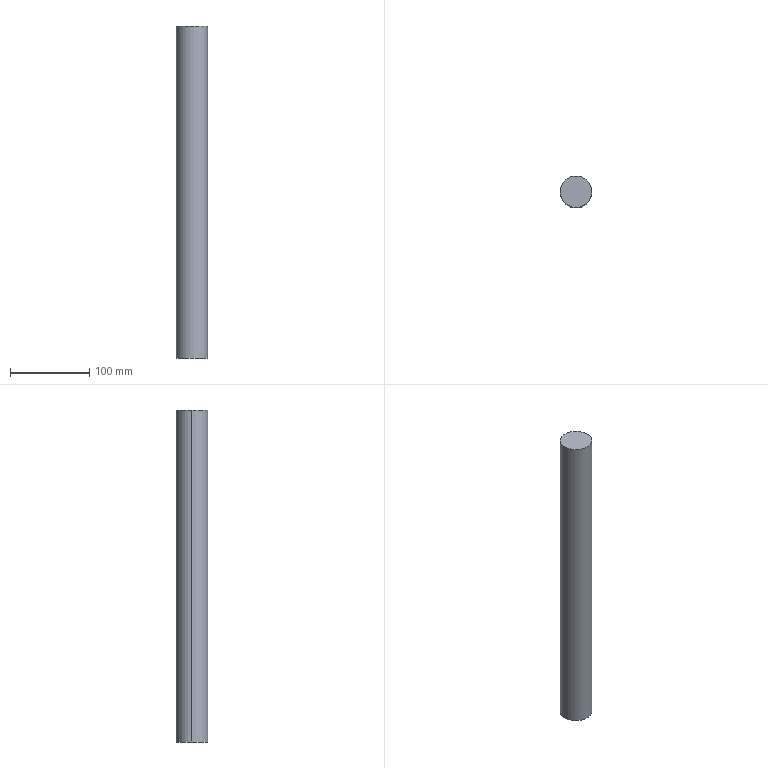Component | SolidWorks | 40Axis-3-8 | 1 solid | 12 faces | box 40 x 40 x 420 mm | volume 526304 mm3 | cylinder 6 | cone 4 | plane 2 | commonest cylinder face diameters 6.8 x4 40 x2 | material 45#
build123d program:
from build123d import *

# Parameters (mm, degrees)
SKETCH1_R             = 20
BOSS_EXTRUDE1_DEPTH   = 210
M8_TAPPED_HOLE1_D     = 6.8
M8_TAPPED_HOLE1_DEPTH = 19.75
M8_TAPPED_HOLE1_TIP   = 2.043


with BuildPart() as part:
    # Sketch1 → Boss-Extrude1 (new, symmetric)
    with BuildSketch(Plane.XY):
        Circle(SKETCH1_R)
    extrude(amount=BOSS_EXTRUDE1_DEPTH, both=True)

    # M8 Tapped Hole1
    with Locations(Plane(origin=(-10, 0, -210), x_dir=(-1, 0, 0), z_dir=(0, 0, -1))):
        with Locations((0, 0), (-20, 0)):
            Hole(M8_TAPPED_HOLE1_D / 2, depth=M8_TAPPED_HOLE1_DEPTH)
            with Locations((0, 0, -(M8_TAPPED_HOLE1_DEPTH + M8_TAPPED_HOLE1_TIP / 2))):  # 118° drill point
                Cone(0, M8_TAPPED_HOLE1_D / 2, M8_TAPPED_HOLE1_TIP, mode=Mode.SUBTRACT)


solid = part.part

# Placed as in the assembly
solid = solid.moved(Location((116.785, -96.917, -574.191), (0, 0, 0)))
STEP:
#1=COLOUR_RGB('',0.7922,0.8196,0.9333);
#2=FILL_AREA_STYLE_COLOUR('',#1);
#3=FILL_AREA_STYLE('',(#2));
#4=SURFACE_STYLE_FILL_AREA(#3);
#5=SURFACE_SIDE_STYLE('',(#4));
#6=SURFACE_STYLE_USAGE(.BOTH.,#5);
#7=PRESENTATION_STYLE_ASSIGNMENT((#6));
#8=CARTESIAN_POINT('',(4.858,-3.816,-30.096));
#9=VERTEX_POINT('',#8);
#10=CARTESIAN_POINT('',(5.125,-3.816,-30.096));
#11=VERTEX_POINT('',#10);
#12=CARTESIAN_POINT('',(4.992,-3.816,-30.096));
#13=DIRECTION('',(0.,0.,-1.));
#14=DIRECTION('',(1.,-0.,0.));
#15=AXIS2_PLACEMENT_3D('',#12,#13,#14);
#16=CIRCLE('',#15,0.1339);
#17=EDGE_CURVE('',#9,#11,#16,.T.);
#18=ORIENTED_EDGE('',*,*,#17,.F.);
#19=CARTESIAN_POINT('',(4.858,-3.816,-30.874));
#20=VERTEX_POINT('',#19);
#21=CARTESIAN_POINT('',(4.858,-3.816,-30.874));
#22=DIRECTION('',(0.,0.,-1.));
#23=VECTOR('',#22,39.37);
#24=LINE('',#21,#23);
#25=EDGE_CURVE('',#9,#20,#24,.T.);
#26=ORIENTED_EDGE('',*,*,#25,.T.);
#27=CARTESIAN_POINT('',(5.125,-3.816,-30.874));
#28=VERTEX_POINT('',#27);
#29=CARTESIAN_POINT('',(4.992,-3.816,-30.874));
#30=DIRECTION('',(0.,0.,-1.));
#31=DIRECTION('',(1.,-0.,0.));
#32=AXIS2_PLACEMENT_3D('',#29,#30,#31);
#33=CIRCLE('',#32,0.1339);
#34=EDGE_CURVE('',#20,#28,#33,.T.);
#35=ORIENTED_EDGE('',*,*,#34,.T.);
#36=CARTESIAN_POINT('',(5.125,-3.816,-30.874));
#37=DIRECTION('',(0.,0.,-1.));
#38=VECTOR('',#37,39.37);
#39=LINE('',#36,#38);
#40=EDGE_CURVE('',#11,#28,#39,.T.);
#41=ORIENTED_EDGE('',*,*,#40,.F.);
#42=EDGE_LOOP('',(#18,#26,#35,#41));
#43=FACE_OUTER_BOUND('',#42,.T.);
#44=CARTESIAN_POINT('',(4.992,-3.816,-30.874));
#45=DIRECTION('',(0.,0.,-1.));
#46=DIRECTION('',(1.,-0.,0.));
#47=AXIS2_PLACEMENT_3D('',#44,#45,#46);
#48=CYLINDRICAL_SURFACE('',#47,0.1339);
#49=ADVANCED_FACE('',(#43),#48,.F.);
#50=CARTESIAN_POINT('',(4.992,-3.816,-30.016));
#51=VERTEX_POINT('',#50);
#52=CARTESIAN_POINT('',(5.125,-3.816,-30.096));
#53=DIRECTION('',(0.8572,-0.,-0.515));
#54=VECTOR('',#53,39.37);
#55=LINE('',#52,#54);
#56=EDGE_CURVE('',#51,#11,#55,.T.);
#57=ORIENTED_EDGE('',*,*,#56,.F.);
#58=CARTESIAN_POINT('',(4.858,-3.816,-30.096));
#59=DIRECTION('',(-0.8572,0.,-0.515));
#60=VECTOR('',#59,39.37);
#61=LINE('',#58,#60);
#62=EDGE_CURVE('',#51,#9,#61,.T.);
#63=ORIENTED_EDGE('',*,*,#62,.T.);
#64=ORIENTED_EDGE('',*,*,#17,.T.);
#65=EDGE_LOOP('',(#57,#63,#64));
#66=FACE_OUTER_BOUND('',#65,.T.);
#67=CARTESIAN_POINT('',(4.992,-3.816,-30.096));
#68=DIRECTION('',(0.,0.,-1.));
#69=DIRECTION('',(1.,-0.,0.));
#70=AXIS2_PLACEMENT_3D('',#67,#68,#69);
#71=CONICAL_SURFACE('',#70,0.1339,1.03);
#72=ADVANCED_FACE('',(#66),#71,.F.);
#73=CARTESIAN_POINT('',(4.07,-3.816,-30.096));
#74=VERTEX_POINT('',#73);
#75=CARTESIAN_POINT('',(4.338,-3.816,-30.096));
#76=VERTEX_POINT('',#75);
#77=CARTESIAN_POINT('',(4.204,-3.816,-30.096));
#78=DIRECTION('',(0.,0.,-1.));
#79=DIRECTION('',(1.,-0.,0.));
#80=AXIS2_PLACEMENT_3D('',#77,#78,#79);
#81=CIRCLE('',#80,0.1339);
#82=EDGE_CURVE('',#74,#76,#81,.T.);
#83=ORIENTED_EDGE('',*,*,#82,.F.);
#84=CARTESIAN_POINT('',(4.07,-3.816,-30.874));
#85=VERTEX_POINT('',#84);
#86=CARTESIAN_POINT('',(4.07,-3.816,-30.874));
#87=DIRECTION('',(0.,0.,-1.));
#88=VECTOR('',#87,39.37);
#89=LINE('',#86,#88);
#90=EDGE_CURVE('',#74,#85,#89,.T.);
#91=ORIENTED_EDGE('',*,*,#90,.T.);
#92=CARTESIAN_POINT('',(4.338,-3.816,-30.874));
#93=VERTEX_POINT('',#92);
#94=CARTESIAN_POINT('',(4.204,-3.816,-30.874));
#95=DIRECTION('',(0.,0.,-1.));
#96=DIRECTION('',(1.,-0.,0.));
#97=AXIS2_PLACEMENT_3D('',#94,#95,#96);
#98=CIRCLE('',#97,0.1339);
#99=EDGE_CURVE('',#85,#93,#98,.T.);
#100=ORIENTED_EDGE('',*,*,#99,.T.);
#101=CARTESIAN_POINT('',(4.338,-3.816,-30.874));
#102=DIRECTION('',(0.,0.,-1.));
#103=VECTOR('',#102,39.37);
#104=LINE('',#101,#103);
#105=EDGE_CURVE('',#76,#93,#104,.T.);
#106=ORIENTED_EDGE('',*,*,#105,.F.);
#107=EDGE_LOOP('',(#83,#91,#100,#106));
#108=FACE_OUTER_BOUND('',#107,.T.);
#109=CARTESIAN_POINT('',(4.204,-3.816,-30.874));
#110=DIRECTION('',(0.,0.,-1.));
#111=DIRECTION('',(1.,-0.,0.));
#112=AXIS2_PLACEMENT_3D('',#109,#110,#111);
#113=CYLINDRICAL_SURFACE('',#112,0.1339);
#114=ADVANCED_FACE('',(#108),#113,.F.);
#115=CARTESIAN_POINT('',(4.204,-3.816,-30.016));
#116=VERTEX_POINT('',#115);
#117=CARTESIAN_POINT('',(4.338,-3.816,-30.096));
#118=DIRECTION('',(0.8572,-0.,-0.515));
#119=VECTOR('',#118,39.37);
#120=LINE('',#117,#119);
#121=EDGE_CURVE('',#116,#76,#120,.T.);
#122=ORIENTED_EDGE('',*,*,#121,.F.);
#123=CARTESIAN_POINT('',(4.07,-3.816,-30.096));
#124=DIRECTION('',(-0.8572,0.,-0.515));
#125=VECTOR('',#124,39.37);
#126=LINE('',#123,#125);
#127=EDGE_CURVE('',#116,#74,#126,.T.);
#128=ORIENTED_EDGE('',*,*,#127,.T.);
#129=ORIENTED_EDGE('',*,*,#82,.T.);
#130=EDGE_LOOP('',(#122,#128,#129));
#131=FACE_OUTER_BOUND('',#130,.T.);
#132=CARTESIAN_POINT('',(4.204,-3.816,-30.096));
#133=DIRECTION('',(0.,0.,-1.));
#134=DIRECTION('',(1.,-0.,0.));
#135=AXIS2_PLACEMENT_3D('',#132,#133,#134);
#136=CONICAL_SURFACE('',#135,0.1339,1.03);
#137=ADVANCED_FACE('',(#131),#136,.F.);
#138=CARTESIAN_POINT('',(3.81,-3.816,-14.338));
#139=VERTEX_POINT('',#138);
#140=CARTESIAN_POINT('',(5.385,-3.816,-14.338));
#141=VERTEX_POINT('',#140);
#142=CARTESIAN_POINT('',(4.598,-3.816,-14.338));
#143=DIRECTION('',(-0.,-0.,1.));
#144=DIRECTION('',(-1.,0.,0.));
#145=AXIS2_PLACEMENT_3D('',#142,#143,#144);
#146=CIRCLE('',#145,0.7874);
#147=EDGE_CURVE('',#139,#141,#146,.T.);
#148=ORIENTED_EDGE('',*,*,#147,.F.);
#149=CARTESIAN_POINT('',(3.81,-3.816,-30.874));
#150=VERTEX_POINT('',#149);
#151=CARTESIAN_POINT('',(3.81,-3.816,-14.338));
#152=DIRECTION('',(0.,0.,-1.));
#153=VECTOR('',#152,39.37);
#154=LINE('',#151,#153);
#155=EDGE_CURVE('',#139,#150,#154,.T.);
#156=ORIENTED_EDGE('',*,*,#155,.T.);
#157=CARTESIAN_POINT('',(5.385,-3.816,-30.874));
#158=VERTEX_POINT('',#157);
#159=CARTESIAN_POINT('',(4.598,-3.816,-30.874));
#160=DIRECTION('',(-0.,-0.,1.));
#161=DIRECTION('',(-1.,0.,0.));
#162=AXIS2_PLACEMENT_3D('',#159,#160,#161);
#163=CIRCLE('',#162,0.7874);
#164=EDGE_CURVE('',#150,#158,#163,.T.);
#165=ORIENTED_EDGE('',*,*,#164,.T.);
#166=CARTESIAN_POINT('',(5.385,-3.816,-14.338));
#167=DIRECTION('',(0.,0.,-1.));
#168=VECTOR('',#167,39.37);
#169=LINE('',#166,#168);
#170=EDGE_CURVE('',#141,#158,#169,.T.);
#171=ORIENTED_EDGE('',*,*,#170,.F.);
#172=EDGE_LOOP('',(#148,#156,#165,#171));
#173=FACE_OUTER_BOUND('',#172,.T.);
#174=CARTESIAN_POINT('',(4.598,-3.816,-14.338));
#175=DIRECTION('',(0.,0.,-1.));
#176=DIRECTION('',(1.,-0.,0.));
#177=AXIS2_PLACEMENT_3D('',#174,#175,#176);
#178=CYLINDRICAL_SURFACE('',#177,0.7874);
#179=ADVANCED_FACE('',(#173),#178,.T.);
#180=ORIENTED_EDGE('',*,*,#155,.F.);
#181=CARTESIAN_POINT('',(4.598,-3.816,-14.338));
#182=DIRECTION('',(-0.,-0.,1.));
#183=DIRECTION('',(-1.,0.,0.));
#184=AXIS2_PLACEMENT_3D('',#181,#182,#183);
#185=CIRCLE('',#184,0.7874);
#186=EDGE_CURVE('',#141,#139,#185,.T.);
#187=ORIENTED_EDGE('',*,*,#186,.F.);
#188=ORIENTED_EDGE('',*,*,#170,.T.);
#189=CARTESIAN_POINT('',(4.598,-3.816,-30.874));
#190=DIRECTION('',(-0.,-0.,1.));
#191=DIRECTION('',(-1.,0.,0.));
#192=AXIS2_PLACEMENT_3D('',#189,#190,#191);
#193=CIRCLE('',#192,0.7874);
#194=EDGE_CURVE('',#158,#150,#193,.T.);
#195=ORIENTED_EDGE('',*,*,#194,.T.);
#196=EDGE_LOOP('',(#180,#187,#188,#195));
#197=FACE_OUTER_BOUND('',#196,.T.);
#198=CARTESIAN_POINT('',(4.598,-3.816,-14.338));
#199=DIRECTION('',(0.,0.,-1.));
#200=DIRECTION('',(1.,-0.,0.));
#201=AXIS2_PLACEMENT_3D('',#198,#199,#200);
#202=CYLINDRICAL_SURFACE('',#201,0.7874);
#203=ADVANCED_FACE('',(#197),#202,.T.);
#204=ORIENTED_EDGE('',*,*,#186,.T.);
#205=ORIENTED_EDGE('',*,*,#147,.T.);
#206=EDGE_LOOP('',(#204,#205));
#207=FACE_OUTER_BOUND('',#206,.T.);
#208=CARTESIAN_POINT('',(4.598,-3.816,-14.338));
#209=DIRECTION('',(-0.,-0.,1.));
#210=DIRECTION('',(-1.,0.,-0.));
#211=AXIS2_PLACEMENT_3D('',#208,#209,#210);
#212=PLANE('',#211);
#213=ADVANCED_FACE('',(#207),#212,.T.);
#214=CARTESIAN_POINT('',(4.992,-3.816,-30.874));
#215=DIRECTION('',(0.,0.,-1.));
#216=DIRECTION('',(1.,-0.,0.));
#217=AXIS2_PLACEMENT_3D('',#214,#215,#216);
#218=CIRCLE('',#217,0.1339);
#219=EDGE_CURVE('',#28,#20,#218,.T.);
#220=ORIENTED_EDGE('',*,*,#219,.F.);
#221=ORIENTED_EDGE('',*,*,#34,.F.);
#222=EDGE_LOOP('',(#220,#221));
#223=FACE_BOUND('',#222,.T.);
#224=CARTESIAN_POINT('',(4.204,-3.816,-30.874));
#225=DIRECTION('',(0.,0.,-1.));
#226=DIRECTION('',(1.,-0.,0.));
#227=AXIS2_PLACEMENT_3D('',#224,#225,#226);
#228=CIRCLE('',#227,0.1339);
#229=EDGE_CURVE('',#93,#85,#228,.T.);
#230=ORIENTED_EDGE('',*,*,#229,.F.);
#231=ORIENTED_EDGE('',*,*,#99,.F.);
#232=EDGE_LOOP('',(#230,#231));
#233=FACE_BOUND('',#232,.T.);
#234=ORIENTED_EDGE('',*,*,#194,.F.);
#235=ORIENTED_EDGE('',*,*,#164,.F.);
#236=EDGE_LOOP('',(#234,#235));
#237=FACE_OUTER_BOUND('',#236,.T.);
#238=CARTESIAN_POINT('',(4.598,-3.816,-30.874));
#239=DIRECTION('',(-0.,-0.,1.));
#240=DIRECTION('',(-1.,0.,-0.));
#241=AXIS2_PLACEMENT_3D('',#238,#239,#240);
#242=PLANE('',#241);
#243=ADVANCED_FACE('',(#223,#233,#237),#242,.F.);
#244=ORIENTED_EDGE('',*,*,#127,.F.);
#245=ORIENTED_EDGE('',*,*,#121,.T.);
#246=CARTESIAN_POINT('',(4.204,-3.816,-30.096));
#247=DIRECTION('',(0.,0.,-1.));
#248=DIRECTION('',(1.,-0.,0.));
#249=AXIS2_PLACEMENT_3D('',#246,#247,#248);
#250=CIRCLE('',#249,0.1339);
#251=EDGE_CURVE('',#76,#74,#250,.T.);
#252=ORIENTED_EDGE('',*,*,#251,.T.);
#253=EDGE_LOOP('',(#244,#245,#252));
#254=FACE_OUTER_BOUND('',#253,.T.);
#255=CARTESIAN_POINT('',(4.204,-3.816,-30.096));
#256=DIRECTION('',(0.,0.,-1.));
#257=DIRECTION('',(1.,-0.,0.));
#258=AXIS2_PLACEMENT_3D('',#255,#256,#257);
#259=CONICAL_SURFACE('',#258,0.1339,1.03);
#260=ADVANCED_FACE('',(#254),#259,.F.);
#261=ORIENTED_EDGE('',*,*,#90,.F.);
#262=ORIENTED_EDGE('',*,*,#251,.F.);
#263=ORIENTED_EDGE('',*,*,#105,.T.);
#264=ORIENTED_EDGE('',*,*,#229,.T.);
#265=EDGE_LOOP('',(#261,#262,#263,#264));
#266=FACE_OUTER_BOUND('',#265,.T.);
#267=CARTESIAN_POINT('',(4.204,-3.816,-30.874));
#268=DIRECTION('',(0.,0.,-1.));
#269=DIRECTION('',(1.,-0.,0.));
#270=AXIS2_PLACEMENT_3D('',#267,#268,#269);
#271=CYLINDRICAL_SURFACE('',#270,0.1339);
#272=ADVANCED_FACE('',(#266),#271,.F.);
#273=ORIENTED_EDGE('',*,*,#62,.F.);
#274=ORIENTED_EDGE('',*,*,#56,.T.);
#275=CARTESIAN_POINT('',(4.992,-3.816,-30.096));
#276=DIRECTION('',(0.,0.,-1.));
#277=DIRECTION('',(1.,-0.,0.));
#278=AXIS2_PLACEMENT_3D('',#275,#276,#277);
#279=CIRCLE('',#278,0.1339);
#280=EDGE_CURVE('',#11,#9,#279,.T.);
#281=ORIENTED_EDGE('',*,*,#280,.T.);
#282=EDGE_LOOP('',(#273,#274,#281));
#283=FACE_OUTER_BOUND('',#282,.T.);
#284=CARTESIAN_POINT('',(4.992,-3.816,-30.096));
#285=DIRECTION('',(0.,0.,-1.));
#286=DIRECTION('',(1.,-0.,0.));
#287=AXIS2_PLACEMENT_3D('',#284,#285,#286);
#288=CONICAL_SURFACE('',#287,0.1339,1.03);
#289=ADVANCED_FACE('',(#283),#288,.F.);
#290=ORIENTED_EDGE('',*,*,#25,.F.);
#291=ORIENTED_EDGE('',*,*,#280,.F.);
#292=ORIENTED_EDGE('',*,*,#40,.T.);
#293=ORIENTED_EDGE('',*,*,#219,.T.);
#294=EDGE_LOOP('',(#290,#291,#292,#293));
#295=FACE_OUTER_BOUND('',#294,.T.);
#296=CARTESIAN_POINT('',(4.992,-3.816,-30.874));
#297=DIRECTION('',(0.,0.,-1.));
#298=DIRECTION('',(1.,-0.,0.));
#299=AXIS2_PLACEMENT_3D('',#296,#297,#298);
#300=CYLINDRICAL_SURFACE('',#299,0.1339);
#301=ADVANCED_FACE('',(#295),#300,.F.);
#302=CLOSED_SHELL('',(#49,#72,#114,#137,#179,#203,#213,#243,#260,#272,#289,#301));
#303=MANIFOLD_SOLID_BREP('',#302);
#304=STYLED_ITEM('',(#7),#303);
#305=(LENGTH_UNIT()NAMED_UNIT(*)SI_UNIT($,.METRE.));
#306=LENGTH_MEASURE_WITH_UNIT(LENGTH_MEASURE(0.0254),#305);
#307=DIMENSIONAL_EXPONENTS(1.,0.,0.,0.,0.,0.,0.);
#308=(CONVERSION_BASED_UNIT('',#306)LENGTH_UNIT()NAMED_UNIT(#307));
#309=UNCERTAINTY_MEASURE_WITH_UNIT(LENGTH_MEASURE(0.00001),#308,'','');
#310=(NAMED_UNIT(*)PLANE_ANGLE_UNIT()SI_UNIT($,.RADIAN.));
#311=(NAMED_UNIT(*)SI_UNIT($,.STERADIAN.)SOLID_ANGLE_UNIT());
#312=(GEOMETRIC_REPRESENTATION_CONTEXT(3)GLOBAL_UNCERTAINTY_ASSIGNED_CONTEXT((#309))GLOBAL_UNIT_ASSIGNED_CONTEXT((#308,#310,#311))REPRESENTATION_CONTEXT('',''));
#313=MECHANICAL_DESIGN_GEOMETRIC_PRESENTATION_REPRESENTATION('',(#304),#312);
#314=PRESENTATION_LAYER_ASSIGNMENT('','',(#304));
#315=CARTESIAN_POINT('',(0.,0.,0.));
#316=DIRECTION('',(0.,0.,1.));
#317=DIRECTION('',(1.,0.,0.));
#318=AXIS2_PLACEMENT_3D('',#315,#316,#317);
#319=(LENGTH_UNIT()NAMED_UNIT(*)SI_UNIT($,.METRE.));
#320=LENGTH_MEASURE_WITH_UNIT(LENGTH_MEASURE(0.0254),#319);
#321=DIMENSIONAL_EXPONENTS(1.,0.,0.,0.,0.,0.,0.);
#322=(CONVERSION_BASED_UNIT('',#320)LENGTH_UNIT()NAMED_UNIT(#321));
#323=UNCERTAINTY_MEASURE_WITH_UNIT(LENGTH_MEASURE(0.00001),#322,'','');
#324=(NAMED_UNIT(*)PLANE_ANGLE_UNIT()SI_UNIT($,.RADIAN.));
#325=(NAMED_UNIT(*)SI_UNIT($,.STERADIAN.)SOLID_ANGLE_UNIT());
#326=(GEOMETRIC_REPRESENTATION_CONTEXT(3)GLOBAL_UNCERTAINTY_ASSIGNED_CONTEXT((#323))GLOBAL_UNIT_ASSIGNED_CONTEXT((#322,#324,#325))REPRESENTATION_CONTEXT('',''));
#327=ADVANCED_BREP_SHAPE_REPRESENTATION('',(#303,#318),#326);